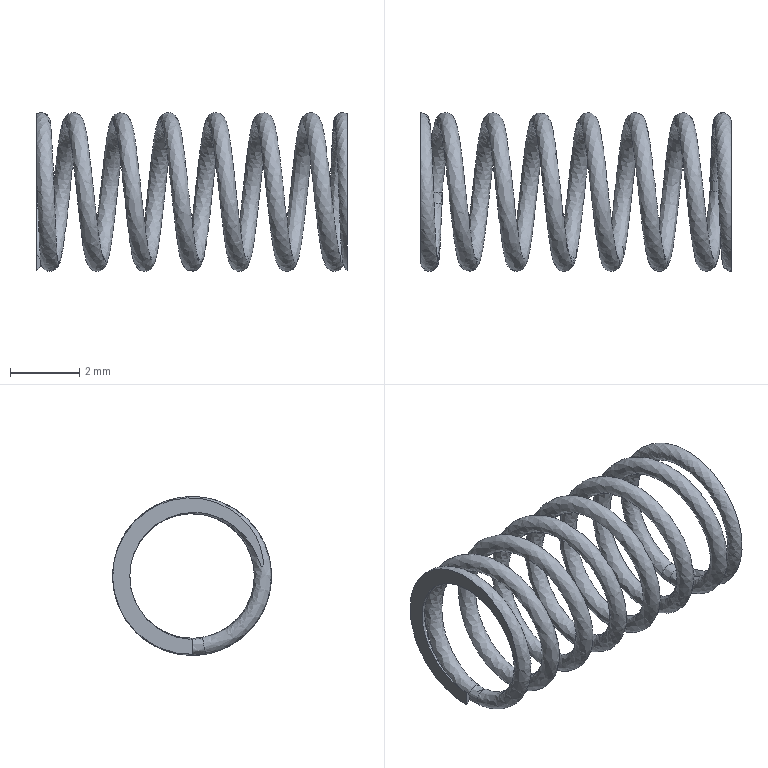Component | NX | SPRING_CYLINDER_COMPRESSION_2 | 1 solid | 9 faces | volume 19 mm3 | spline 5 | plane 4